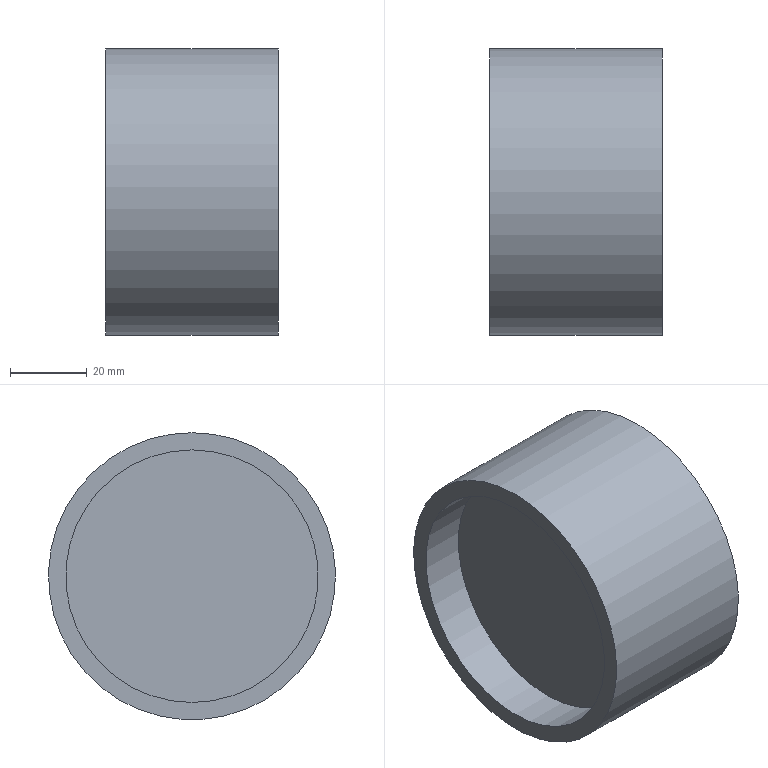Component | NX | CLOCKHAND1 | 1 solid | 7 faces | box 45 x 75 x 75 mm | volume 116695 mm3 | plane 4 | cylinder 3 | commonest cylinder face diameters 66 x2 75 x1
STEP:
#1=CARTESIAN_POINT('',(0.,0.,0.));
#2=DIRECTION('',(0.,0.,1.));
#3=DIRECTION('',(1.,0.,0.));
#4=AXIS2_PLACEMENT_3D('',#1,#2,#3);
#5=CARTESIAN_POINT('',(-148.42,281.257,63.472));
#6=VERTEX_POINT('',#5);
#7=CARTESIAN_POINT('',(-148.42,281.257,30.472));
#8=DIRECTION('',(1.,0.,0.));
#9=DIRECTION('',(0.,0.,1.));
#10=AXIS2_PLACEMENT_3D('',#7,#8,#9);
#11=CIRCLE('',#10,33.);
#12=CARTESIAN_POINT('',(-148.42,281.257,30.472));
#13=DIRECTION('',(-1.,0.,0.));
#14=DIRECTION('',(0.,0.,1.));
#15=AXIS2_PLACEMENT_3D('',#12,#13,#14);
#16=PLANE('',#15);
#17=CARTESIAN_POINT('',(33.,0.));
#18=CARTESIAN_POINT('',(33.,-57.158));
#19=CARTESIAN_POINT('',(-16.5,-28.579));
#20=CARTESIAN_POINT('',(-66.,-0.));
#21=CARTESIAN_POINT('',(-16.5,28.579));
#22=CARTESIAN_POINT('',(33.,57.158));
#23=CARTESIAN_POINT('',(33.,0.));
#24=(BOUNDED_CURVE()B_SPLINE_CURVE(2,(#17,#18,#19,#20,#21,#22,#23),.UNSPECIFIED.,.T.,.F.)B_SPLINE_CURVE_WITH_KNOTS((1,2,2,2,2,1),(-2.094,0.,2.094,4.189,6.283,8.378),.UNSPECIFIED.)CURVE()GEOMETRIC_REPRESENTATION_ITEM()RATIONAL_B_SPLINE_CURVE((1.,0.5,1.,0.5,1.,0.5,1.))REPRESENTATION_ITEM(''));
#25=(GEOMETRIC_REPRESENTATION_CONTEXT(2)PARAMETRIC_REPRESENTATION_CONTEXT()REPRESENTATION_CONTEXT('',''));
#26=DEFINITIONAL_REPRESENTATION('',(#24),#25);
#27=PCURVE('',#16,#26);
#28=CARTESIAN_POINT('',(-148.42,281.257,30.472));
#29=DIRECTION('',(1.,0.,0.));
#30=DIRECTION('',(0.,0.,1.));
#31=AXIS2_PLACEMENT_3D('',#28,#29,#30);
#32=CYLINDRICAL_SURFACE('',#31,33.);
#33=CARTESIAN_POINT('',(0.,0.));
#34=DIRECTION('',(1.,0.));
#35=VECTOR('',#34,1.);
#36=LINE('',#33,#35);
#37=(GEOMETRIC_REPRESENTATION_CONTEXT(2)PARAMETRIC_REPRESENTATION_CONTEXT()REPRESENTATION_CONTEXT('',''));
#38=DEFINITIONAL_REPRESENTATION('',(#36),#37);
#39=PCURVE('',#32,#38);
#40=SURFACE_CURVE('',#11,(#27,#39),.PCURVE_S1.);
#41=EDGE_CURVE('',#6,#6,#40,.T.);
#42=ORIENTED_EDGE('',*,*,#41,.T.);
#43=EDGE_LOOP('',(#42));
#44=FACE_BOUND('',#43,.T.);
#45=CARTESIAN_POINT('',(-148.42,281.257,67.972));
#46=VERTEX_POINT('',#45);
#47=CARTESIAN_POINT('',(-148.42,281.257,30.472));
#48=DIRECTION('',(1.,0.,0.));
#49=DIRECTION('',(0.,0.,1.));
#50=AXIS2_PLACEMENT_3D('',#47,#48,#49);
#51=CIRCLE('',#50,37.5);
#52=CARTESIAN_POINT('',(37.5,0.));
#53=CARTESIAN_POINT('',(37.5,-64.952));
#54=CARTESIAN_POINT('',(-18.75,-32.476));
#55=CARTESIAN_POINT('',(-75.,-0.));
#56=CARTESIAN_POINT('',(-18.75,32.476));
#57=CARTESIAN_POINT('',(37.5,64.952));
#58=CARTESIAN_POINT('',(37.5,0.));
#59=(BOUNDED_CURVE()B_SPLINE_CURVE(2,(#52,#53,#54,#55,#56,#57,#58),.UNSPECIFIED.,.T.,.F.)B_SPLINE_CURVE_WITH_KNOTS((1,2,2,2,2,1),(-2.094,0.,2.094,4.189,6.283,8.378),.UNSPECIFIED.)CURVE()GEOMETRIC_REPRESENTATION_ITEM()RATIONAL_B_SPLINE_CURVE((1.,0.5,1.,0.5,1.,0.5,1.))REPRESENTATION_ITEM(''));
#60=(GEOMETRIC_REPRESENTATION_CONTEXT(2)PARAMETRIC_REPRESENTATION_CONTEXT()REPRESENTATION_CONTEXT('',''));
#61=DEFINITIONAL_REPRESENTATION('',(#59),#60);
#62=PCURVE('',#16,#61);
#63=CARTESIAN_POINT('',(-103.42,281.257,30.472));
#64=DIRECTION('',(-1.,0.,0.));
#65=DIRECTION('',(0.,0.,1.));
#66=AXIS2_PLACEMENT_3D('',#63,#64,#65);
#67=CYLINDRICAL_SURFACE('',#66,37.5);
#68=CARTESIAN_POINT('',(6.283,45.));
#69=DIRECTION('',(-1.,0.));
#70=VECTOR('',#69,1.);
#71=LINE('',#68,#70);
#72=(GEOMETRIC_REPRESENTATION_CONTEXT(2)PARAMETRIC_REPRESENTATION_CONTEXT()REPRESENTATION_CONTEXT('',''));
#73=DEFINITIONAL_REPRESENTATION('',(#71),#72);
#74=PCURVE('',#67,#73);
#75=SURFACE_CURVE('',#51,(#62,#74),.PCURVE_S1.);
#76=EDGE_CURVE('',#46,#46,#75,.T.);
#77=ORIENTED_EDGE('',*,*,#76,.F.);
#78=EDGE_LOOP('',(#77));
#79=FACE_BOUND('',#78,.T.);
#80=ADVANCED_FACE('',(#44,#79),#16,.T.);
#81=CARTESIAN_POINT('',(-103.42,281.257,63.472));
#82=VERTEX_POINT('',#81);
#83=CARTESIAN_POINT('',(-103.42,281.257,30.472));
#84=DIRECTION('',(-1.,0.,0.));
#85=DIRECTION('',(0.,0.,1.));
#86=AXIS2_PLACEMENT_3D('',#83,#84,#85);
#87=CIRCLE('',#86,33.);
#88=CARTESIAN_POINT('',(-103.42,281.257,30.472));
#89=DIRECTION('',(1.,0.,0.));
#90=DIRECTION('',(0.,0.,-1.));
#91=AXIS2_PLACEMENT_3D('',#88,#89,#90);
#92=PLANE('',#91);
#93=CARTESIAN_POINT('',(-33.,0.));
#94=CARTESIAN_POINT('',(-33.,57.158));
#95=CARTESIAN_POINT('',(16.5,28.579));
#96=CARTESIAN_POINT('',(66.,0.));
#97=CARTESIAN_POINT('',(16.5,-28.579));
#98=CARTESIAN_POINT('',(-33.,-57.158));
#99=CARTESIAN_POINT('',(-33.,0.));
#100=(BOUNDED_CURVE()B_SPLINE_CURVE(2,(#93,#94,#95,#96,#97,#98,#99),.UNSPECIFIED.,.T.,.F.)B_SPLINE_CURVE_WITH_KNOTS((1,2,2,2,2,1),(-2.094,0.,2.094,4.189,6.283,8.378),.UNSPECIFIED.)CURVE()GEOMETRIC_REPRESENTATION_ITEM()RATIONAL_B_SPLINE_CURVE((1.,0.5,1.,0.5,1.,0.5,1.))REPRESENTATION_ITEM(''));
#101=(GEOMETRIC_REPRESENTATION_CONTEXT(2)PARAMETRIC_REPRESENTATION_CONTEXT()REPRESENTATION_CONTEXT('',''));
#102=DEFINITIONAL_REPRESENTATION('',(#100),#101);
#103=PCURVE('',#92,#102);
#104=CARTESIAN_POINT('',(-103.42,281.257,30.472));
#105=DIRECTION('',(-1.,0.,0.));
#106=DIRECTION('',(0.,0.,1.));
#107=AXIS2_PLACEMENT_3D('',#104,#105,#106);
#108=CYLINDRICAL_SURFACE('',#107,33.);
#109=CARTESIAN_POINT('',(0.,0.));
#110=DIRECTION('',(1.,0.));
#111=VECTOR('',#110,1.);
#112=LINE('',#109,#111);
#113=(GEOMETRIC_REPRESENTATION_CONTEXT(2)PARAMETRIC_REPRESENTATION_CONTEXT()REPRESENTATION_CONTEXT('',''));
#114=DEFINITIONAL_REPRESENTATION('',(#112),#113);
#115=PCURVE('',#108,#114);
#116=SURFACE_CURVE('',#87,(#103,#115),.PCURVE_S1.);
#117=EDGE_CURVE('',#82,#82,#116,.T.);
#118=ORIENTED_EDGE('',*,*,#117,.T.);
#119=EDGE_LOOP('',(#118));
#120=FACE_BOUND('',#119,.T.);
#121=CARTESIAN_POINT('',(-103.42,281.257,67.972));
#122=VERTEX_POINT('',#121);
#123=CARTESIAN_POINT('',(-103.42,281.257,30.472));
#124=DIRECTION('',(-1.,0.,0.));
#125=DIRECTION('',(0.,0.,1.));
#126=AXIS2_PLACEMENT_3D('',#123,#124,#125);
#127=CIRCLE('',#126,37.5);
#128=CARTESIAN_POINT('',(-37.5,0.));
#129=CARTESIAN_POINT('',(-37.5,64.952));
#130=CARTESIAN_POINT('',(18.75,32.476));
#131=CARTESIAN_POINT('',(75.,0.));
#132=CARTESIAN_POINT('',(18.75,-32.476));
#133=CARTESIAN_POINT('',(-37.5,-64.952));
#134=CARTESIAN_POINT('',(-37.5,0.));
#135=(BOUNDED_CURVE()B_SPLINE_CURVE(2,(#128,#129,#130,#131,#132,#133,#134),.UNSPECIFIED.,.T.,.F.)B_SPLINE_CURVE_WITH_KNOTS((1,2,2,2,2,1),(-2.094,0.,2.094,4.189,6.283,8.378),.UNSPECIFIED.)CURVE()GEOMETRIC_REPRESENTATION_ITEM()RATIONAL_B_SPLINE_CURVE((1.,0.5,1.,0.5,1.,0.5,1.))REPRESENTATION_ITEM(''));
#136=(GEOMETRIC_REPRESENTATION_CONTEXT(2)PARAMETRIC_REPRESENTATION_CONTEXT()REPRESENTATION_CONTEXT('',''));
#137=DEFINITIONAL_REPRESENTATION('',(#135),#136);
#138=PCURVE('',#92,#137);
#139=CARTESIAN_POINT('',(0.,0.));
#140=DIRECTION('',(1.,0.));
#141=VECTOR('',#140,1.);
#142=LINE('',#139,#141);
#143=(GEOMETRIC_REPRESENTATION_CONTEXT(2)PARAMETRIC_REPRESENTATION_CONTEXT()REPRESENTATION_CONTEXT('',''));
#144=DEFINITIONAL_REPRESENTATION('',(#142),#143);
#145=PCURVE('',#67,#144);
#146=SURFACE_CURVE('',#127,(#138,#145),.PCURVE_S1.);
#147=EDGE_CURVE('',#122,#122,#146,.T.);
#148=ORIENTED_EDGE('',*,*,#147,.F.);
#149=EDGE_LOOP('',(#148));
#150=FACE_BOUND('',#149,.T.);
#151=ADVANCED_FACE('',(#120,#150),#92,.T.);
#152=ORIENTED_EDGE('',*,*,#76,.T.);
#153=CARTESIAN_POINT('',(-103.42,281.257,67.972));
#154=CARTESIAN_POINT('',(-148.42,281.257,67.972));
#155=B_SPLINE_CURVE_WITH_KNOTS('',1,(#153,#154),.UNSPECIFIED.,.F.,.F.,(2,2),(0.,45.),.PIECEWISE_BEZIER_KNOTS.);
#156=CARTESIAN_POINT('',(0.,0.));
#157=DIRECTION('',(0.,1.));
#158=VECTOR('',#157,1.);
#159=LINE('',#156,#158);
#160=(GEOMETRIC_REPRESENTATION_CONTEXT(2)PARAMETRIC_REPRESENTATION_CONTEXT()REPRESENTATION_CONTEXT('',''));
#161=DEFINITIONAL_REPRESENTATION('',(#159),#160);
#162=PCURVE('',#67,#161);
#163=CARTESIAN_POINT('',(6.283,0.));
#164=DIRECTION('',(0.,1.));
#165=VECTOR('',#164,1.);
#166=LINE('',#163,#165);
#167=(GEOMETRIC_REPRESENTATION_CONTEXT(2)PARAMETRIC_REPRESENTATION_CONTEXT()REPRESENTATION_CONTEXT('',''));
#168=DEFINITIONAL_REPRESENTATION('',(#166),#167);
#169=PCURVE('',#67,#168);
#170=SEAM_CURVE('',#155,(#162,#169),.PCURVE_S1.);
#171=EDGE_CURVE('',#122,#46,#170,.T.);
#172=ORIENTED_EDGE('',*,*,#171,.F.);
#173=ORIENTED_EDGE('',*,*,#147,.T.);
#174=ORIENTED_EDGE('',*,*,#171,.T.);
#175=EDGE_LOOP('',(#152,#172,#173,#174));
#176=FACE_BOUND('',#175,.T.);
#177=ADVANCED_FACE('',(#176),#67,.T.);
#178=CARTESIAN_POINT('',(-115.42,281.257,63.472));
#179=VERTEX_POINT('',#178);
#180=CARTESIAN_POINT('',(-115.42,281.257,30.472));
#181=DIRECTION('',(-1.,0.,0.));
#182=DIRECTION('',(0.,0.,1.));
#183=AXIS2_PLACEMENT_3D('',#180,#181,#182);
#184=CIRCLE('',#183,33.);
#185=CARTESIAN_POINT('',(-115.42,281.257,30.472));
#186=DIRECTION('',(-1.,0.,0.));
#187=DIRECTION('',(0.,0.,1.));
#188=AXIS2_PLACEMENT_3D('',#185,#186,#187);
#189=PLANE('',#188);
#190=CARTESIAN_POINT('',(0.,0.));
#191=DIRECTION('',(1.,0.));
#192=AXIS2_PLACEMENT_2D('',#190,#191);
#193=CIRCLE('',#192,33.);
#194=(GEOMETRIC_REPRESENTATION_CONTEXT(2)PARAMETRIC_REPRESENTATION_CONTEXT()REPRESENTATION_CONTEXT('',''));
#195=DEFINITIONAL_REPRESENTATION('',(#193),#194);
#196=PCURVE('',#189,#195);
#197=CARTESIAN_POINT('',(0.,12.));
#198=DIRECTION('',(1.,0.));
#199=VECTOR('',#198,1.);
#200=LINE('',#197,#199);
#201=(GEOMETRIC_REPRESENTATION_CONTEXT(2)PARAMETRIC_REPRESENTATION_CONTEXT()REPRESENTATION_CONTEXT('',''));
#202=DEFINITIONAL_REPRESENTATION('',(#200),#201);
#203=PCURVE('',#108,#202);
#204=SURFACE_CURVE('',#184,(#196,#203),.PCURVE_S1.);
#205=EDGE_CURVE('',#179,#179,#204,.T.);
#206=ORIENTED_EDGE('',*,*,#205,.F.);
#207=EDGE_LOOP('',(#206));
#208=FACE_BOUND('',#207,.T.);
#209=ADVANCED_FACE('',(#208),#189,.F.);
#210=ORIENTED_EDGE('',*,*,#205,.F.);
#211=CARTESIAN_POINT('',(-103.42,281.257,63.472));
#212=CARTESIAN_POINT('',(-115.42,281.257,63.472));
#213=B_SPLINE_CURVE_WITH_KNOTS('',1,(#211,#212),.UNSPECIFIED.,.F.,.F.,(2,2),(0.,12.),.PIECEWISE_BEZIER_KNOTS.);
#214=CARTESIAN_POINT('',(0.,0.));
#215=DIRECTION('',(0.,1.));
#216=VECTOR('',#215,1.);
#217=LINE('',#214,#216);
#218=(GEOMETRIC_REPRESENTATION_CONTEXT(2)PARAMETRIC_REPRESENTATION_CONTEXT()REPRESENTATION_CONTEXT('',''));
#219=DEFINITIONAL_REPRESENTATION('',(#217),#218);
#220=PCURVE('',#108,#219);
#221=CARTESIAN_POINT('',(6.283,0.));
#222=DIRECTION('',(0.,1.));
#223=VECTOR('',#222,1.);
#224=LINE('',#221,#223);
#225=(GEOMETRIC_REPRESENTATION_CONTEXT(2)PARAMETRIC_REPRESENTATION_CONTEXT()REPRESENTATION_CONTEXT('',''));
#226=DEFINITIONAL_REPRESENTATION('',(#224),#225);
#227=PCURVE('',#108,#226);
#228=SEAM_CURVE('',#213,(#220,#227),.PCURVE_S1.);
#229=EDGE_CURVE('',#82,#179,#228,.T.);
#230=ORIENTED_EDGE('',*,*,#229,.F.);
#231=ORIENTED_EDGE('',*,*,#117,.T.);
#232=ORIENTED_EDGE('',*,*,#229,.T.);
#233=EDGE_LOOP('',(#210,#230,#231,#232));
#234=FACE_BOUND('',#233,.F.);
#235=ADVANCED_FACE('',(#234),#108,.F.);
#236=CARTESIAN_POINT('',(-136.42,281.257,63.472));
#237=VERTEX_POINT('',#236);
#238=CARTESIAN_POINT('',(-136.42,281.257,30.472));
#239=DIRECTION('',(1.,0.,0.));
#240=DIRECTION('',(0.,0.,1.));
#241=AXIS2_PLACEMENT_3D('',#238,#239,#240);
#242=CIRCLE('',#241,33.);
#243=CARTESIAN_POINT('',(-136.42,281.257,30.472));
#244=DIRECTION('',(1.,0.,0.));
#245=DIRECTION('',(0.,0.,-1.));
#246=AXIS2_PLACEMENT_3D('',#243,#244,#245);
#247=PLANE('',#246);
#248=CARTESIAN_POINT('',(0.,0.));
#249=DIRECTION('',(-1.,0.));
#250=AXIS2_PLACEMENT_2D('',#248,#249);
#251=CIRCLE('',#250,33.);
#252=(GEOMETRIC_REPRESENTATION_CONTEXT(2)PARAMETRIC_REPRESENTATION_CONTEXT()REPRESENTATION_CONTEXT('',''));
#253=DEFINITIONAL_REPRESENTATION('',(#251),#252);
#254=PCURVE('',#247,#253);
#255=CARTESIAN_POINT('',(0.,12.));
#256=DIRECTION('',(1.,0.));
#257=VECTOR('',#256,1.);
#258=LINE('',#255,#257);
#259=(GEOMETRIC_REPRESENTATION_CONTEXT(2)PARAMETRIC_REPRESENTATION_CONTEXT()REPRESENTATION_CONTEXT('',''));
#260=DEFINITIONAL_REPRESENTATION('',(#258),#259);
#261=PCURVE('',#32,#260);
#262=SURFACE_CURVE('',#242,(#254,#261),.PCURVE_S1.);
#263=EDGE_CURVE('',#237,#237,#262,.T.);
#264=ORIENTED_EDGE('',*,*,#263,.F.);
#265=EDGE_LOOP('',(#264));
#266=FACE_BOUND('',#265,.T.);
#267=ADVANCED_FACE('',(#266),#247,.F.);
#268=ORIENTED_EDGE('',*,*,#263,.F.);
#269=CARTESIAN_POINT('',(-148.42,281.257,63.472));
#270=CARTESIAN_POINT('',(-136.42,281.257,63.472));
#271=B_SPLINE_CURVE_WITH_KNOTS('',1,(#269,#270),.UNSPECIFIED.,.F.,.F.,(2,2),(0.,12.),.PIECEWISE_BEZIER_KNOTS.);
#272=CARTESIAN_POINT('',(0.,0.));
#273=DIRECTION('',(0.,1.));
#274=VECTOR('',#273,1.);
#275=LINE('',#272,#274);
#276=(GEOMETRIC_REPRESENTATION_CONTEXT(2)PARAMETRIC_REPRESENTATION_CONTEXT()REPRESENTATION_CONTEXT('',''));
#277=DEFINITIONAL_REPRESENTATION('',(#275),#276);
#278=PCURVE('',#32,#277);
#279=CARTESIAN_POINT('',(6.283,0.));
#280=DIRECTION('',(0.,1.));
#281=VECTOR('',#280,1.);
#282=LINE('',#279,#281);
#283=(GEOMETRIC_REPRESENTATION_CONTEXT(2)PARAMETRIC_REPRESENTATION_CONTEXT()REPRESENTATION_CONTEXT('',''));
#284=DEFINITIONAL_REPRESENTATION('',(#282),#283);
#285=PCURVE('',#32,#284);
#286=SEAM_CURVE('',#271,(#278,#285),.PCURVE_S1.);
#287=EDGE_CURVE('',#6,#237,#286,.T.);
#288=ORIENTED_EDGE('',*,*,#287,.F.);
#289=ORIENTED_EDGE('',*,*,#41,.T.);
#290=ORIENTED_EDGE('',*,*,#287,.T.);
#291=EDGE_LOOP('',(#268,#288,#289,#290));
#292=FACE_BOUND('',#291,.F.);
#293=ADVANCED_FACE('',(#292),#32,.F.);
#294=CLOSED_SHELL('',(#80,#151,#177,#209,#235,#267,#293));
#295=MANIFOLD_SOLID_BREP('',#294);
#296=(LENGTH_UNIT()NAMED_UNIT(*)SI_UNIT(.MILLI.,.METRE.));
#297=UNCERTAINTY_MEASURE_WITH_UNIT(LENGTH_MEASURE(0.00001),#296,'','');
#298=(NAMED_UNIT(*)PLANE_ANGLE_UNIT()SI_UNIT($,.RADIAN.));
#299=(NAMED_UNIT(*)SI_UNIT($,.STERADIAN.)SOLID_ANGLE_UNIT());
#300=(GEOMETRIC_REPRESENTATION_CONTEXT(3)GLOBAL_UNCERTAINTY_ASSIGNED_CONTEXT((#297))GLOBAL_UNIT_ASSIGNED_CONTEXT((#296,#298,#299))REPRESENTATION_CONTEXT('',''));
#301=ADVANCED_BREP_SHAPE_REPRESENTATION('',(#4,#295),#300);